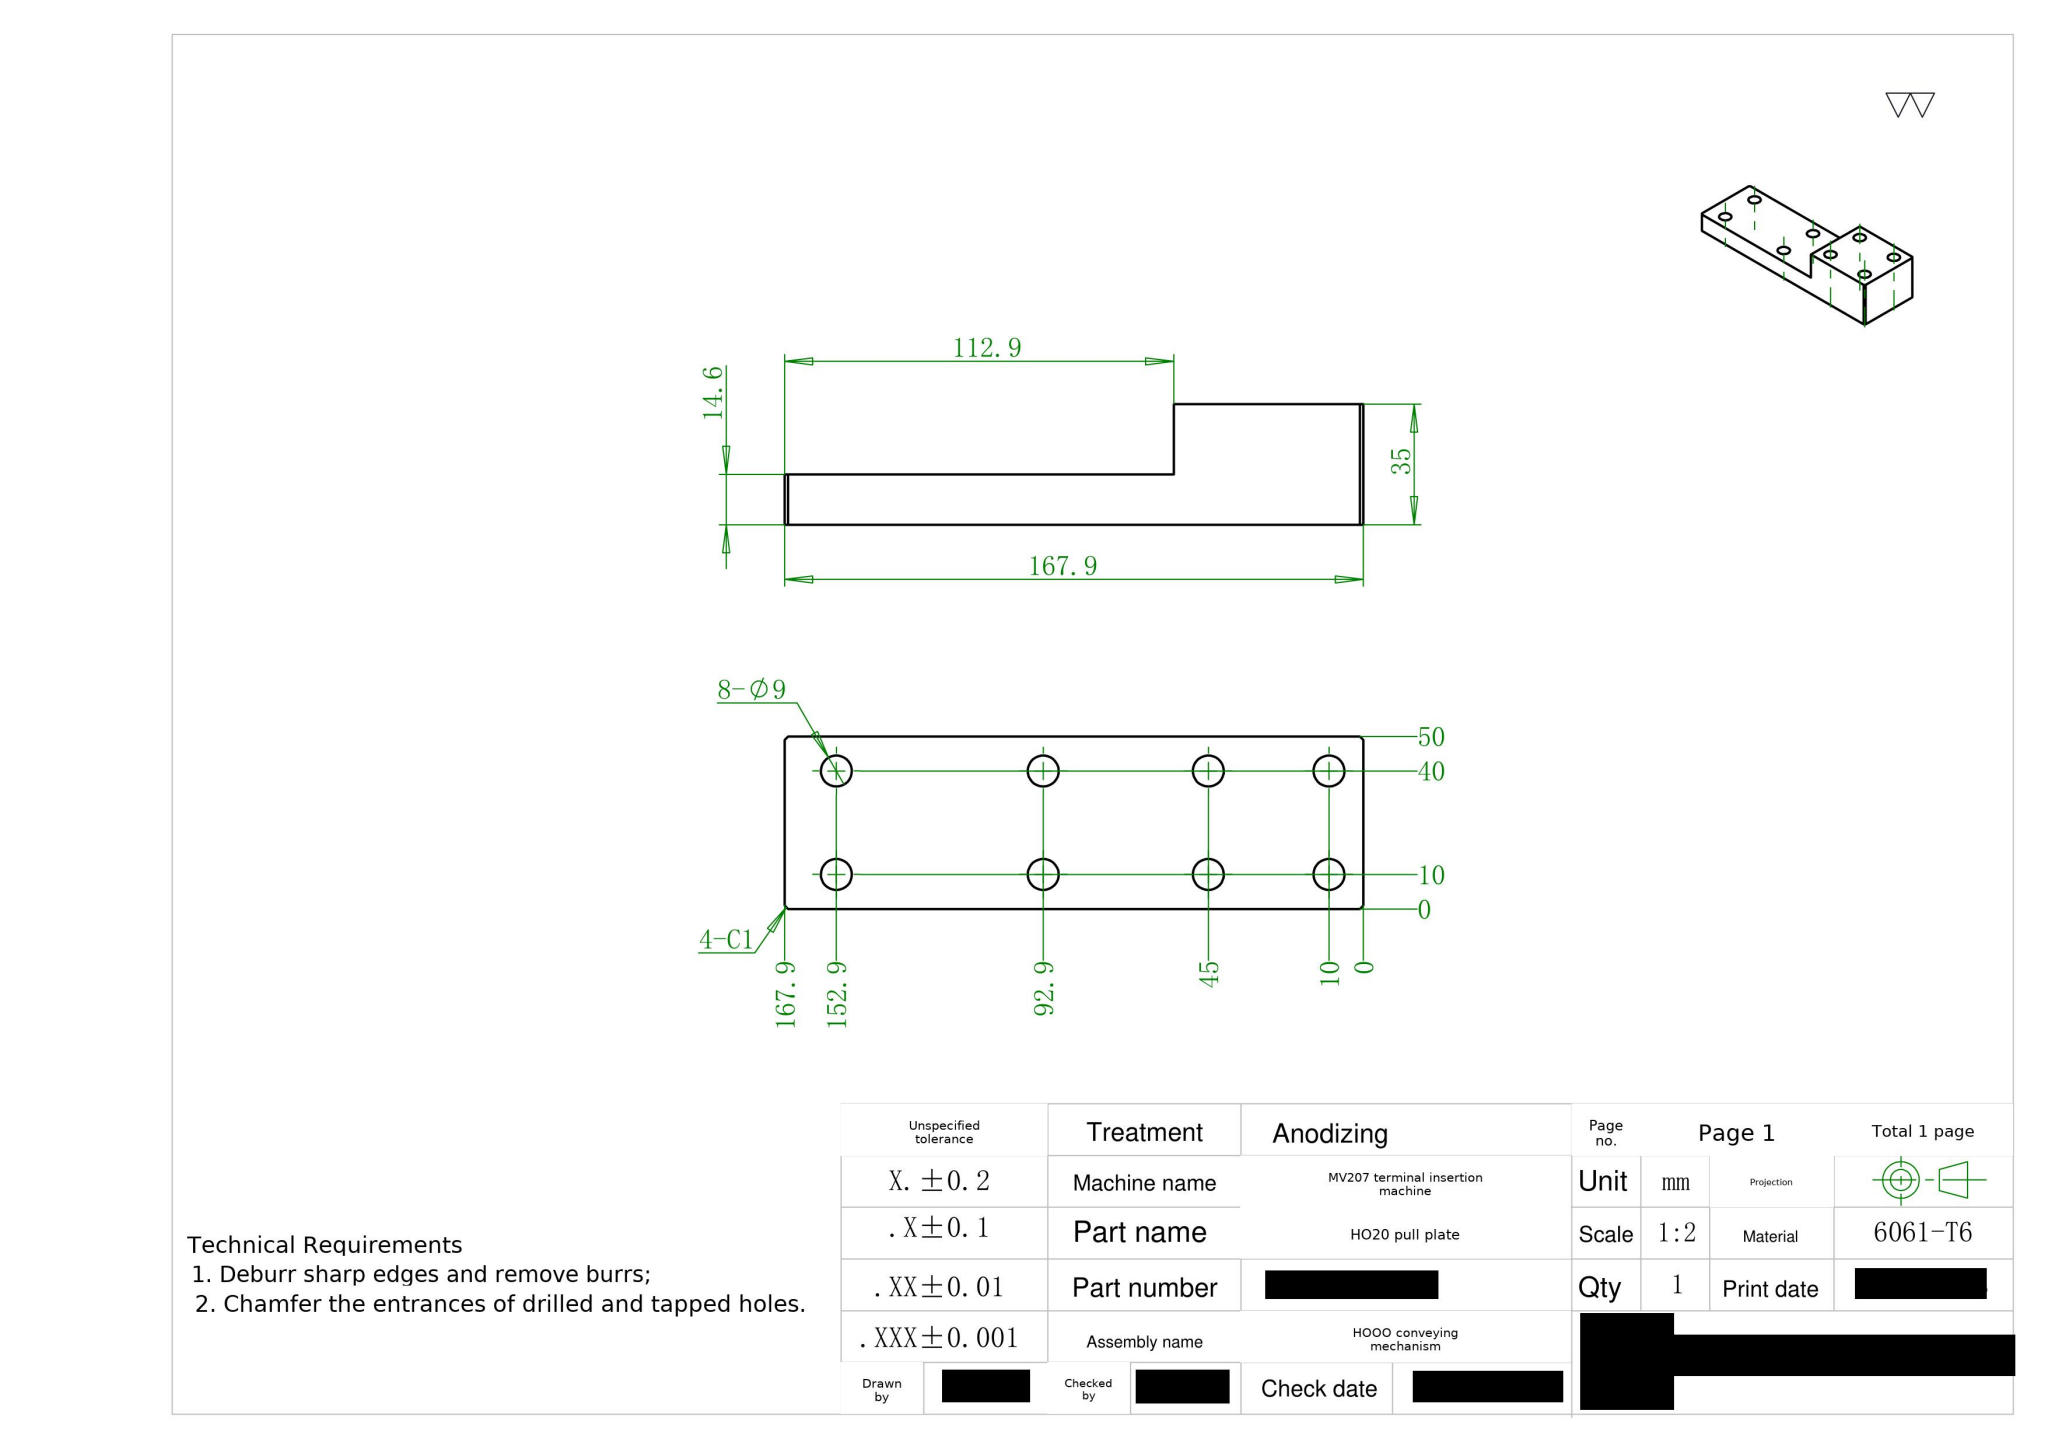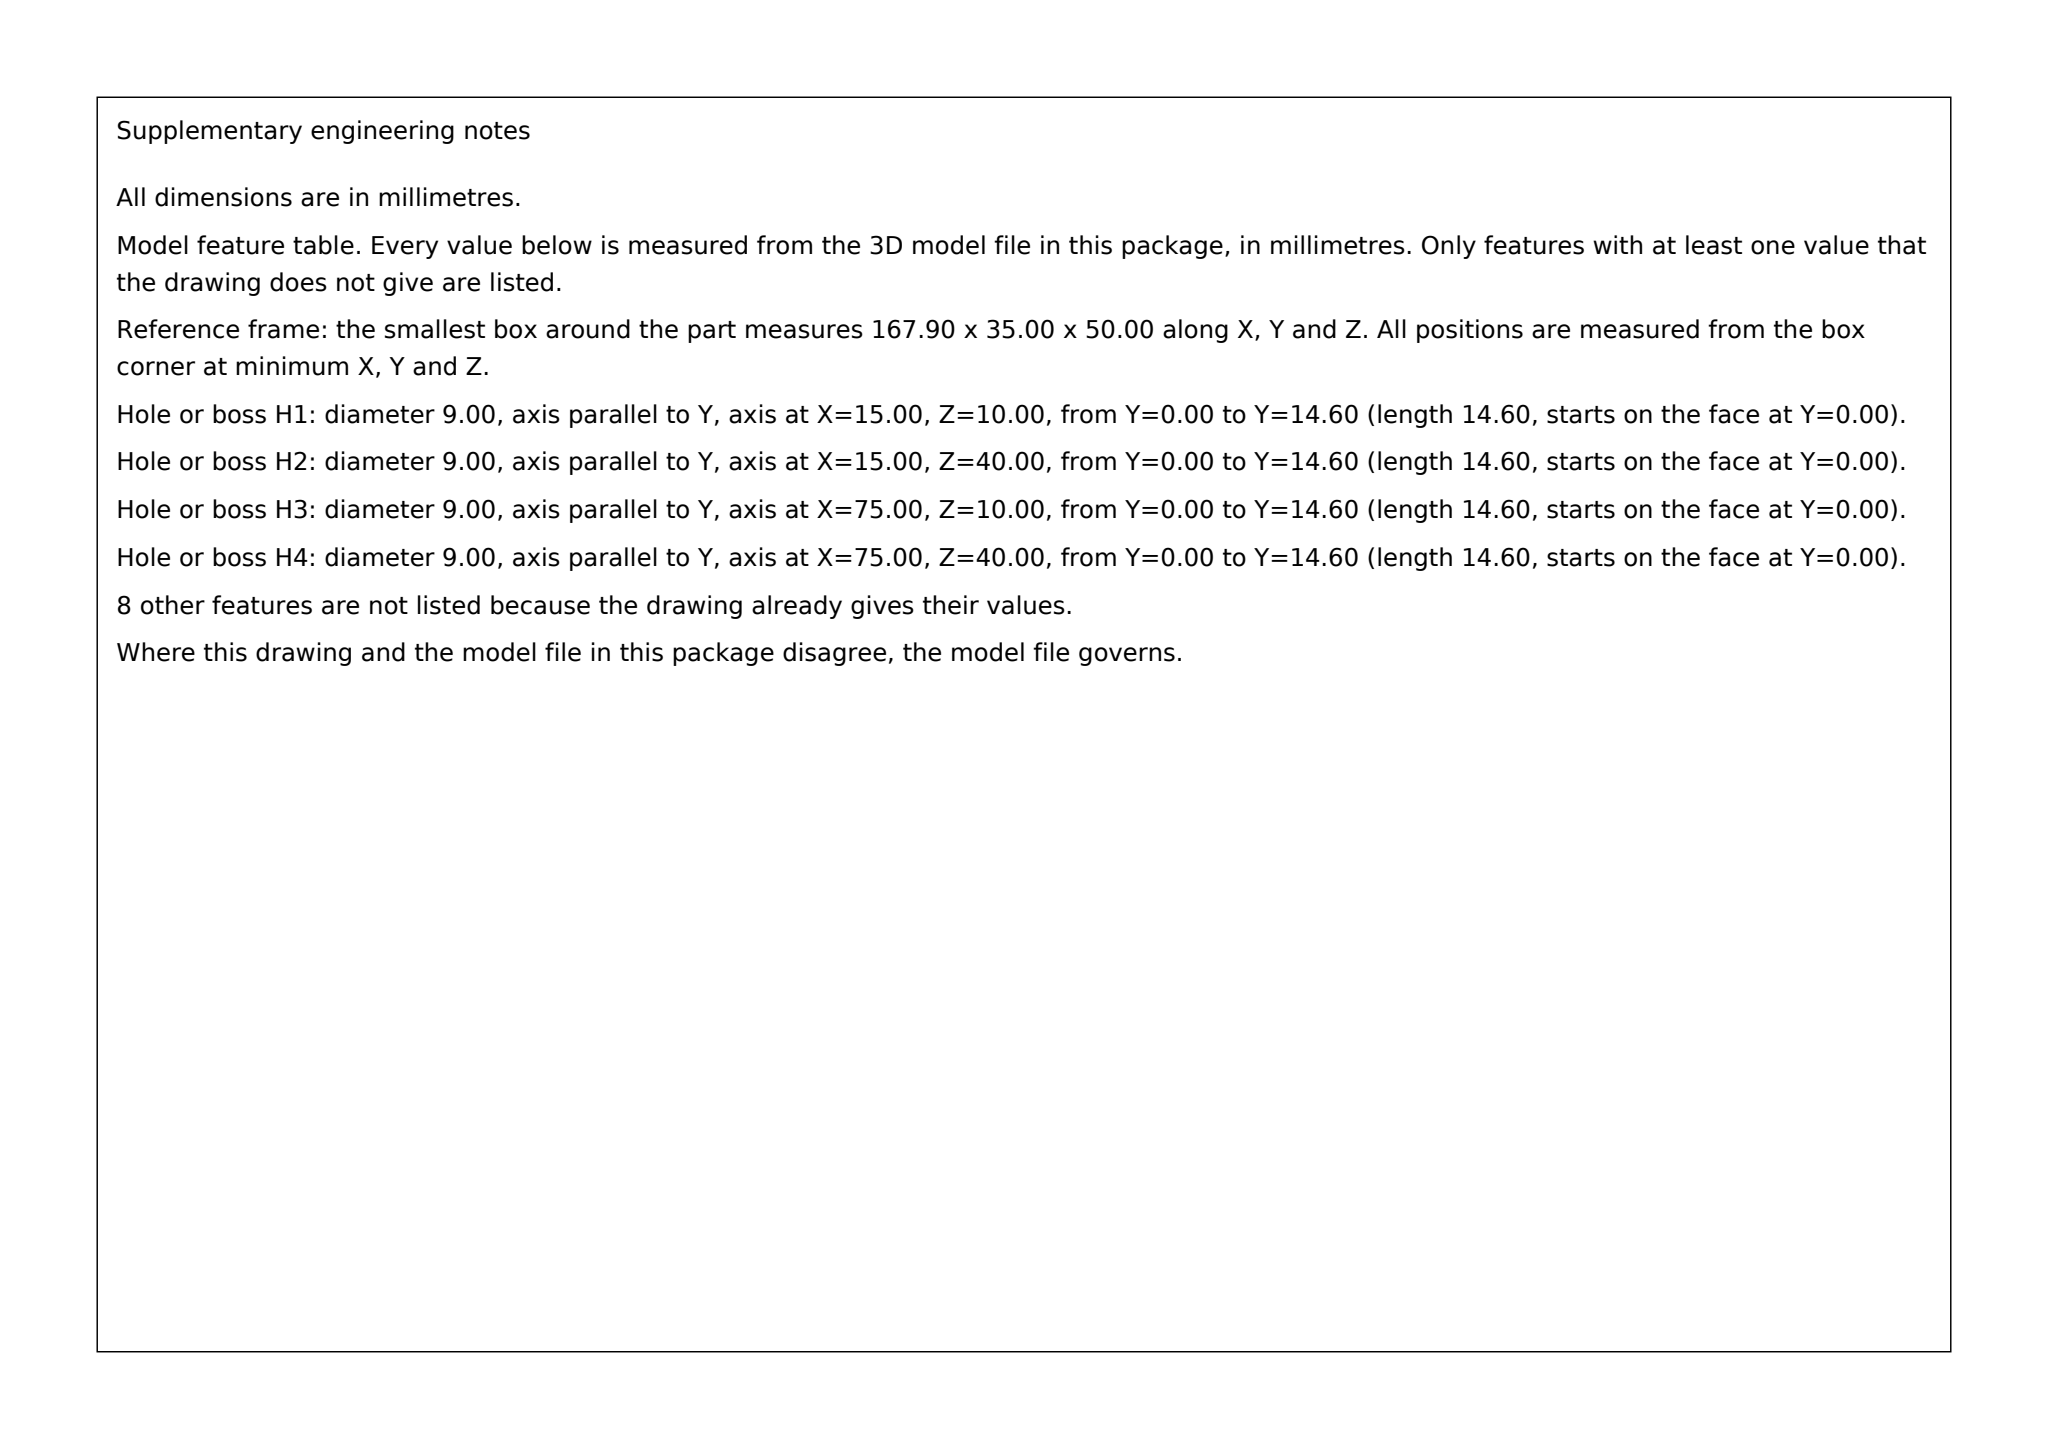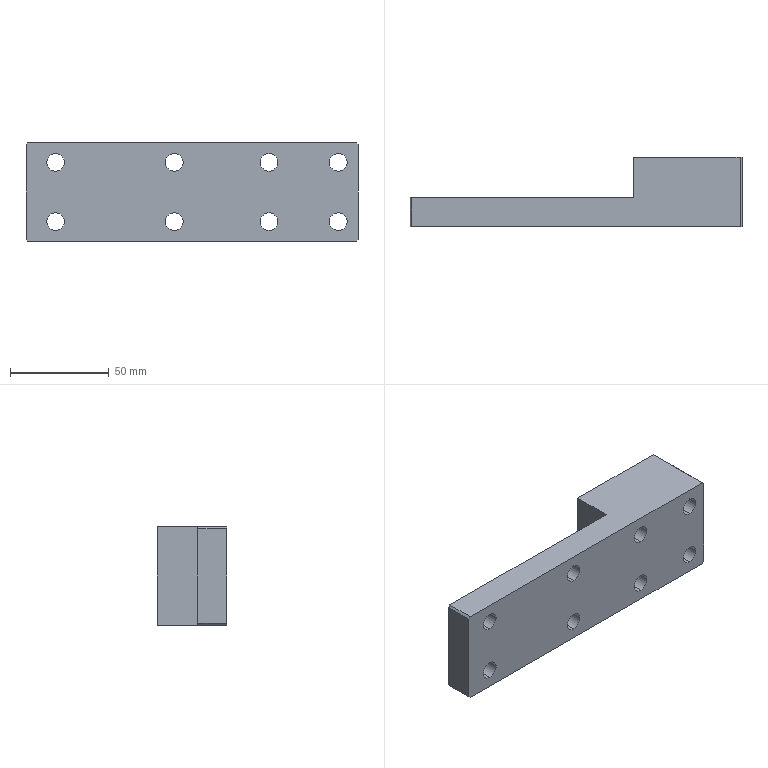Part | SolidWorks | mm | material 6061-T6 | 1 solid | 28 faces | box 167.9 x 35 x 50 mm | volume 165996 mm3 | cylinder 16 | plane 12 | commonest cylinder face diameters 9 x16
build123d program:
from build123d import *

# Parameters (mm, degrees)
BOSS_EXTRUDE1_DEPTH      = 50
F_9_0_9_DIAMETER_HOLE1_D = 9
CHAMFER1_SIZE            = 1


with BuildPart() as part:
    # Sketch1 → Boss-Extrude1 (new body)
    with BuildSketch(Plane.XY):
        Polygon((0, 0), (0, 14.6), (112.9, 14.6), (112.9, 35), (167.9, 35), (167.9, 0), align=None)
    extrude(amount=BOSS_EXTRUDE1_DEPTH)

    # 9.0 _9_ Diameter Hole1 (through all)
    with Locations(Plane(origin=(0, 0, 0), x_dir=(-1, 0, 0), z_dir=(0, -1, 0))):
        with Locations((-15, -40), (-75, -40), (-122.9, -40), (-157.9, -40), (-157.9, -10), (-122.9, -10), (-75, -10), (-15, -10)):
            Hole(F_9_0_9_DIAMETER_HOLE1_D / 2)

    # Chamfer1
    chamfer1_edges = [part.edges().sort_by_distance(p)[0] for p in [
        (0, 7.3, 50),
        (0, 7.3, 0),
        (167.9, 17.5, 50),
        (167.9, 17.5, 0),
    ]]
    chamfer(chamfer1_edges, length=CHAMFER1_SIZE)


solid = part.part